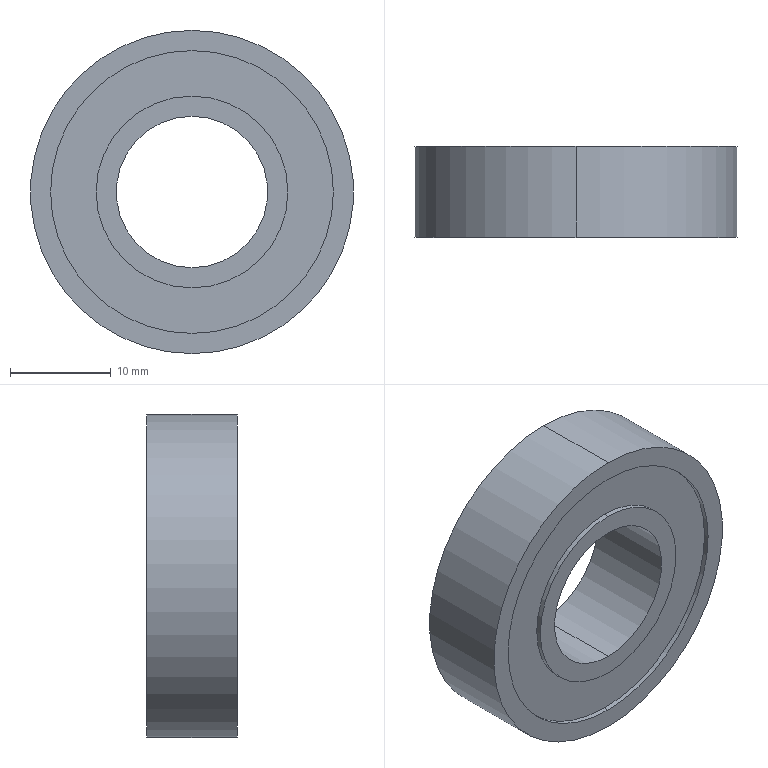Component | SolidWorks | 8TC-A15004-83-00-16_6002-2 | 1 solid | 18 faces | box 32 x 9 x 32 mm | volume 5316 mm3 | cylinder 12 | plane 6 | commonest cylinder face diameters 28 x4 19 x4 32 x2 15 x2
build123d program:
from build123d import *


with BuildPart() as part:
    # Sketch1 → Revolve1 (revolve)
    with BuildSketch(Plane(origin=(0, 0, 0), x_dir=(1, 0, 0), z_dir=(0, 1, 0)), mode=Mode.PRIVATE) as revolve1_sk:
        Polygon((-16, -4.5), (-16, 4.5), (-14, 4.5), (-14, 4), (-9.5, 4), (-9.5, 4.5), (-7.5, 4.5), (-7.5, -4.5), (-9.5, -4.5), (-9.5, -4), (-14, -4), (-14, -4.5), align=None)
    revolve(revolve1_sk.sketch.rotate(Axis((0, 0, 0), (0, 0, -1)), 180), axis=Axis((0, 0, 0), (0, 0, -1)))


solid = part.part

# Placed as in the assembly
solid = solid.moved(Location((40, 233, 60), (90, 0, 0)))
STEP:
#1=COLOUR_RGB('',0.7922,0.8196,0.9333);
#2=FILL_AREA_STYLE_COLOUR('',#1);
#3=FILL_AREA_STYLE('',(#2));
#4=SURFACE_STYLE_FILL_AREA(#3);
#5=SURFACE_SIDE_STYLE('',(#4));
#6=SURFACE_STYLE_USAGE(.BOTH.,#5);
#7=PRESENTATION_STYLE_ASSIGNMENT((#6));
#8=CARTESIAN_POINT('',(1.575,9.35,2.992));
#9=VERTEX_POINT('',#8);
#10=CARTESIAN_POINT('',(1.575,9.35,1.732));
#11=VERTEX_POINT('',#10);
#12=CARTESIAN_POINT('',(1.575,9.35,2.362));
#13=DIRECTION('',(-0.,-1.,0.));
#14=DIRECTION('',(0.,0.,1.));
#15=AXIS2_PLACEMENT_3D('',#12,#13,#14);
#16=CIRCLE('',#15,0.6299);
#17=EDGE_CURVE('',#9,#11,#16,.T.);
#18=ORIENTED_EDGE('',*,*,#17,.T.);
#19=CARTESIAN_POINT('',(1.575,8.996,1.732));
#20=VERTEX_POINT('',#19);
#21=CARTESIAN_POINT('',(1.575,9.173,1.732));
#22=DIRECTION('',(-0.,-1.,0.));
#23=VECTOR('',#22,39.37);
#24=LINE('',#21,#23);
#25=EDGE_CURVE('',#11,#20,#24,.T.);
#26=ORIENTED_EDGE('',*,*,#25,.T.);
#27=CARTESIAN_POINT('',(1.575,8.996,2.992));
#28=VERTEX_POINT('',#27);
#29=CARTESIAN_POINT('',(1.575,8.996,2.362));
#30=DIRECTION('',(-0.,-1.,0.));
#31=DIRECTION('',(0.,0.,1.));
#32=AXIS2_PLACEMENT_3D('',#29,#30,#31);
#33=CIRCLE('',#32,0.6299);
#34=EDGE_CURVE('',#28,#20,#33,.T.);
#35=ORIENTED_EDGE('',*,*,#34,.F.);
#36=CARTESIAN_POINT('',(1.575,9.173,2.992));
#37=DIRECTION('',(-0.,-1.,0.));
#38=VECTOR('',#37,39.37);
#39=LINE('',#36,#38);
#40=EDGE_CURVE('',#9,#28,#39,.T.);
#41=ORIENTED_EDGE('',*,*,#40,.F.);
#42=EDGE_LOOP('',(#18,#26,#35,#41));
#43=FACE_OUTER_BOUND('',#42,.T.);
#44=CARTESIAN_POINT('',(1.575,9.173,2.362));
#45=DIRECTION('',(-0.,-1.,0.));
#46=DIRECTION('',(0.,0.,1.));
#47=AXIS2_PLACEMENT_3D('',#44,#45,#46);
#48=CYLINDRICAL_SURFACE('',#47,0.6299);
#49=ADVANCED_FACE('',(#43),#48,.T.);
#50=CARTESIAN_POINT('',(1.575,9.016,1.811));
#51=VERTEX_POINT('',#50);
#52=CARTESIAN_POINT('',(1.575,9.016,2.913));
#53=VERTEX_POINT('',#52);
#54=CARTESIAN_POINT('',(1.575,9.016,2.362));
#55=DIRECTION('',(-0.,-1.,0.));
#56=DIRECTION('',(0.,0.,1.));
#57=AXIS2_PLACEMENT_3D('',#54,#55,#56);
#58=CIRCLE('',#57,0.5512);
#59=EDGE_CURVE('',#51,#53,#58,.T.);
#60=ORIENTED_EDGE('',*,*,#59,.F.);
#61=CARTESIAN_POINT('',(1.575,8.996,1.811));
#62=VERTEX_POINT('',#61);
#63=CARTESIAN_POINT('',(1.575,9.173,1.811));
#64=DIRECTION('',(-0.,-1.,0.));
#65=VECTOR('',#64,39.37);
#66=LINE('',#63,#65);
#67=EDGE_CURVE('',#51,#62,#66,.T.);
#68=ORIENTED_EDGE('',*,*,#67,.T.);
#69=CARTESIAN_POINT('',(1.575,8.996,2.913));
#70=VERTEX_POINT('',#69);
#71=CARTESIAN_POINT('',(1.575,8.996,2.362));
#72=DIRECTION('',(-0.,-1.,0.));
#73=DIRECTION('',(0.,0.,1.));
#74=AXIS2_PLACEMENT_3D('',#71,#72,#73);
#75=CIRCLE('',#74,0.5512);
#76=EDGE_CURVE('',#62,#70,#75,.T.);
#77=ORIENTED_EDGE('',*,*,#76,.T.);
#78=CARTESIAN_POINT('',(1.575,9.173,2.913));
#79=DIRECTION('',(-0.,-1.,0.));
#80=VECTOR('',#79,39.37);
#81=LINE('',#78,#80);
#82=EDGE_CURVE('',#53,#70,#81,.T.);
#83=ORIENTED_EDGE('',*,*,#82,.F.);
#84=EDGE_LOOP('',(#60,#68,#77,#83));
#85=FACE_OUTER_BOUND('',#84,.T.);
#86=CARTESIAN_POINT('',(1.575,9.173,2.362));
#87=DIRECTION('',(-0.,-1.,0.));
#88=DIRECTION('',(0.,0.,1.));
#89=AXIS2_PLACEMENT_3D('',#86,#87,#88);
#90=CYLINDRICAL_SURFACE('',#89,0.5512);
#91=ADVANCED_FACE('',(#85),#90,.F.);
#92=CARTESIAN_POINT('',(1.575,9.016,2.736));
#93=VERTEX_POINT('',#92);
#94=CARTESIAN_POINT('',(1.575,9.016,1.988));
#95=VERTEX_POINT('',#94);
#96=CARTESIAN_POINT('',(1.575,9.016,2.362));
#97=DIRECTION('',(-0.,-1.,0.));
#98=DIRECTION('',(0.,0.,1.));
#99=AXIS2_PLACEMENT_3D('',#96,#97,#98);
#100=CIRCLE('',#99,0.374);
#101=EDGE_CURVE('',#93,#95,#100,.T.);
#102=ORIENTED_EDGE('',*,*,#101,.T.);
#103=CARTESIAN_POINT('',(1.575,8.996,1.988));
#104=VERTEX_POINT('',#103);
#105=CARTESIAN_POINT('',(1.575,9.173,1.988));
#106=DIRECTION('',(-0.,-1.,0.));
#107=VECTOR('',#106,39.37);
#108=LINE('',#105,#107);
#109=EDGE_CURVE('',#95,#104,#108,.T.);
#110=ORIENTED_EDGE('',*,*,#109,.T.);
#111=CARTESIAN_POINT('',(1.575,8.996,2.736));
#112=VERTEX_POINT('',#111);
#113=CARTESIAN_POINT('',(1.575,8.996,2.362));
#114=DIRECTION('',(-0.,-1.,0.));
#115=DIRECTION('',(0.,0.,1.));
#116=AXIS2_PLACEMENT_3D('',#113,#114,#115);
#117=CIRCLE('',#116,0.374);
#118=EDGE_CURVE('',#112,#104,#117,.T.);
#119=ORIENTED_EDGE('',*,*,#118,.F.);
#120=CARTESIAN_POINT('',(1.575,9.173,2.736));
#121=DIRECTION('',(-0.,-1.,0.));
#122=VECTOR('',#121,39.37);
#123=LINE('',#120,#122);
#124=EDGE_CURVE('',#93,#112,#123,.T.);
#125=ORIENTED_EDGE('',*,*,#124,.F.);
#126=EDGE_LOOP('',(#102,#110,#119,#125));
#127=FACE_OUTER_BOUND('',#126,.T.);
#128=CARTESIAN_POINT('',(1.575,9.173,2.362));
#129=DIRECTION('',(-0.,-1.,0.));
#130=DIRECTION('',(0.,0.,1.));
#131=AXIS2_PLACEMENT_3D('',#128,#129,#130);
#132=CYLINDRICAL_SURFACE('',#131,0.374);
#133=ADVANCED_FACE('',(#127),#132,.T.);
#134=CARTESIAN_POINT('',(1.575,9.35,2.067));
#135=VERTEX_POINT('',#134);
#136=CARTESIAN_POINT('',(1.575,9.35,2.657));
#137=VERTEX_POINT('',#136);
#138=CARTESIAN_POINT('',(1.575,9.35,2.362));
#139=DIRECTION('',(-0.,-1.,0.));
#140=DIRECTION('',(0.,0.,1.));
#141=AXIS2_PLACEMENT_3D('',#138,#139,#140);
#142=CIRCLE('',#141,0.2953);
#143=EDGE_CURVE('',#135,#137,#142,.T.);
#144=ORIENTED_EDGE('',*,*,#143,.F.);
#145=CARTESIAN_POINT('',(1.575,8.996,2.067));
#146=VERTEX_POINT('',#145);
#147=CARTESIAN_POINT('',(1.575,9.173,2.067));
#148=DIRECTION('',(-0.,-1.,0.));
#149=VECTOR('',#148,39.37);
#150=LINE('',#147,#149);
#151=EDGE_CURVE('',#135,#146,#150,.T.);
#152=ORIENTED_EDGE('',*,*,#151,.T.);
#153=CARTESIAN_POINT('',(1.575,8.996,2.657));
#154=VERTEX_POINT('',#153);
#155=CARTESIAN_POINT('',(1.575,8.996,2.362));
#156=DIRECTION('',(-0.,-1.,0.));
#157=DIRECTION('',(0.,0.,1.));
#158=AXIS2_PLACEMENT_3D('',#155,#156,#157);
#159=CIRCLE('',#158,0.2953);
#160=EDGE_CURVE('',#146,#154,#159,.T.);
#161=ORIENTED_EDGE('',*,*,#160,.T.);
#162=CARTESIAN_POINT('',(1.575,9.173,2.657));
#163=DIRECTION('',(-0.,-1.,0.));
#164=VECTOR('',#163,39.37);
#165=LINE('',#162,#164);
#166=EDGE_CURVE('',#137,#154,#165,.T.);
#167=ORIENTED_EDGE('',*,*,#166,.F.);
#168=EDGE_LOOP('',(#144,#152,#161,#167));
#169=FACE_OUTER_BOUND('',#168,.T.);
#170=CARTESIAN_POINT('',(1.575,9.173,2.362));
#171=DIRECTION('',(-0.,-1.,0.));
#172=DIRECTION('',(0.,0.,1.));
#173=AXIS2_PLACEMENT_3D('',#170,#171,#172);
#174=CYLINDRICAL_SURFACE('',#173,0.2953);
#175=ADVANCED_FACE('',(#169),#174,.F.);
#176=CARTESIAN_POINT('',(1.575,9.35,2.736));
#177=VERTEX_POINT('',#176);
#178=CARTESIAN_POINT('',(1.575,9.35,1.988));
#179=VERTEX_POINT('',#178);
#180=CARTESIAN_POINT('',(1.575,9.35,2.362));
#181=DIRECTION('',(-0.,-1.,0.));
#182=DIRECTION('',(0.,0.,1.));
#183=AXIS2_PLACEMENT_3D('',#180,#181,#182);
#184=CIRCLE('',#183,0.374);
#185=EDGE_CURVE('',#177,#179,#184,.T.);
#186=ORIENTED_EDGE('',*,*,#185,.T.);
#187=CARTESIAN_POINT('',(1.575,9.331,1.988));
#188=VERTEX_POINT('',#187);
#189=CARTESIAN_POINT('',(1.575,9.173,1.988));
#190=DIRECTION('',(-0.,-1.,0.));
#191=VECTOR('',#190,39.37);
#192=LINE('',#189,#191);
#193=EDGE_CURVE('',#179,#188,#192,.T.);
#194=ORIENTED_EDGE('',*,*,#193,.T.);
#195=CARTESIAN_POINT('',(1.575,9.331,2.736));
#196=VERTEX_POINT('',#195);
#197=CARTESIAN_POINT('',(1.575,9.331,2.362));
#198=DIRECTION('',(-0.,-1.,0.));
#199=DIRECTION('',(0.,0.,1.));
#200=AXIS2_PLACEMENT_3D('',#197,#198,#199);
#201=CIRCLE('',#200,0.374);
#202=EDGE_CURVE('',#196,#188,#201,.T.);
#203=ORIENTED_EDGE('',*,*,#202,.F.);
#204=CARTESIAN_POINT('',(1.575,9.173,2.736));
#205=DIRECTION('',(-0.,-1.,0.));
#206=VECTOR('',#205,39.37);
#207=LINE('',#204,#206);
#208=EDGE_CURVE('',#177,#196,#207,.T.);
#209=ORIENTED_EDGE('',*,*,#208,.F.);
#210=EDGE_LOOP('',(#186,#194,#203,#209));
#211=FACE_OUTER_BOUND('',#210,.T.);
#212=CARTESIAN_POINT('',(1.575,9.173,2.362));
#213=DIRECTION('',(-0.,-1.,0.));
#214=DIRECTION('',(0.,0.,1.));
#215=AXIS2_PLACEMENT_3D('',#212,#213,#214);
#216=CYLINDRICAL_SURFACE('',#215,0.374);
#217=ADVANCED_FACE('',(#211),#216,.T.);
#218=CARTESIAN_POINT('',(1.575,9.35,1.811));
#219=VERTEX_POINT('',#218);
#220=CARTESIAN_POINT('',(1.575,9.35,2.913));
#221=VERTEX_POINT('',#220);
#222=CARTESIAN_POINT('',(1.575,9.35,2.362));
#223=DIRECTION('',(-0.,-1.,0.));
#224=DIRECTION('',(0.,0.,1.));
#225=AXIS2_PLACEMENT_3D('',#222,#223,#224);
#226=CIRCLE('',#225,0.5512);
#227=EDGE_CURVE('',#219,#221,#226,.T.);
#228=ORIENTED_EDGE('',*,*,#227,.F.);
#229=CARTESIAN_POINT('',(1.575,9.331,1.811));
#230=VERTEX_POINT('',#229);
#231=CARTESIAN_POINT('',(1.575,9.173,1.811));
#232=DIRECTION('',(-0.,-1.,0.));
#233=VECTOR('',#232,39.37);
#234=LINE('',#231,#233);
#235=EDGE_CURVE('',#219,#230,#234,.T.);
#236=ORIENTED_EDGE('',*,*,#235,.T.);
#237=CARTESIAN_POINT('',(1.575,9.331,2.913));
#238=VERTEX_POINT('',#237);
#239=CARTESIAN_POINT('',(1.575,9.331,2.362));
#240=DIRECTION('',(-0.,-1.,0.));
#241=DIRECTION('',(0.,0.,1.));
#242=AXIS2_PLACEMENT_3D('',#239,#240,#241);
#243=CIRCLE('',#242,0.5512);
#244=EDGE_CURVE('',#230,#238,#243,.T.);
#245=ORIENTED_EDGE('',*,*,#244,.T.);
#246=CARTESIAN_POINT('',(1.575,9.173,2.913));
#247=DIRECTION('',(-0.,-1.,0.));
#248=VECTOR('',#247,39.37);
#249=LINE('',#246,#248);
#250=EDGE_CURVE('',#221,#238,#249,.T.);
#251=ORIENTED_EDGE('',*,*,#250,.F.);
#252=EDGE_LOOP('',(#228,#236,#245,#251));
#253=FACE_OUTER_BOUND('',#252,.T.);
#254=CARTESIAN_POINT('',(1.575,9.173,2.362));
#255=DIRECTION('',(-0.,-1.,0.));
#256=DIRECTION('',(0.,0.,1.));
#257=AXIS2_PLACEMENT_3D('',#254,#255,#256);
#258=CYLINDRICAL_SURFACE('',#257,0.5512);
#259=ADVANCED_FACE('',(#253),#258,.F.);
#260=ORIENTED_EDGE('',*,*,#17,.F.);
#261=CARTESIAN_POINT('',(1.575,9.35,2.362));
#262=DIRECTION('',(-0.,-1.,0.));
#263=DIRECTION('',(0.,0.,1.));
#264=AXIS2_PLACEMENT_3D('',#261,#262,#263);
#265=CIRCLE('',#264,0.6299);
#266=EDGE_CURVE('',#11,#9,#265,.T.);
#267=ORIENTED_EDGE('',*,*,#266,.F.);
#268=EDGE_LOOP('',(#260,#267));
#269=FACE_OUTER_BOUND('',#268,.T.);
#270=CARTESIAN_POINT('',(1.575,9.35,2.362));
#271=DIRECTION('',(-0.,-1.,0.));
#272=DIRECTION('',(0.,0.,1.));
#273=AXIS2_PLACEMENT_3D('',#270,#271,#272);
#274=CIRCLE('',#273,0.5512);
#275=EDGE_CURVE('',#221,#219,#274,.T.);
#276=ORIENTED_EDGE('',*,*,#275,.T.);
#277=ORIENTED_EDGE('',*,*,#227,.T.);
#278=EDGE_LOOP('',(#276,#277));
#279=FACE_BOUND('',#278,.T.);
#280=CARTESIAN_POINT('',(1.575,9.35,1.732));
#281=DIRECTION('',(-0.,-1.,0.));
#282=DIRECTION('',(0.,0.,1.));
#283=AXIS2_PLACEMENT_3D('',#280,#281,#282);
#284=PLANE('',#283);
#285=ADVANCED_FACE('',(#269,#279),#284,.F.);
#286=ORIENTED_EDGE('',*,*,#235,.F.);
#287=ORIENTED_EDGE('',*,*,#275,.F.);
#288=ORIENTED_EDGE('',*,*,#250,.T.);
#289=CARTESIAN_POINT('',(1.575,9.331,2.362));
#290=DIRECTION('',(-0.,-1.,0.));
#291=DIRECTION('',(0.,0.,1.));
#292=AXIS2_PLACEMENT_3D('',#289,#290,#291);
#293=CIRCLE('',#292,0.5512);
#294=EDGE_CURVE('',#238,#230,#293,.T.);
#295=ORIENTED_EDGE('',*,*,#294,.T.);
#296=EDGE_LOOP('',(#286,#287,#288,#295));
#297=FACE_OUTER_BOUND('',#296,.T.);
#298=CARTESIAN_POINT('',(1.575,9.173,2.362));
#299=DIRECTION('',(-0.,-1.,0.));
#300=DIRECTION('',(0.,0.,1.));
#301=AXIS2_PLACEMENT_3D('',#298,#299,#300);
#302=CYLINDRICAL_SURFACE('',#301,0.5512);
#303=ADVANCED_FACE('',(#297),#302,.F.);
#304=ORIENTED_EDGE('',*,*,#294,.F.);
#305=ORIENTED_EDGE('',*,*,#244,.F.);
#306=EDGE_LOOP('',(#304,#305));
#307=FACE_OUTER_BOUND('',#306,.T.);
#308=ORIENTED_EDGE('',*,*,#202,.T.);
#309=CARTESIAN_POINT('',(1.575,9.331,2.362));
#310=DIRECTION('',(-0.,-1.,0.));
#311=DIRECTION('',(0.,0.,1.));
#312=AXIS2_PLACEMENT_3D('',#309,#310,#311);
#313=CIRCLE('',#312,0.374);
#314=EDGE_CURVE('',#188,#196,#313,.T.);
#315=ORIENTED_EDGE('',*,*,#314,.T.);
#316=EDGE_LOOP('',(#308,#315));
#317=FACE_BOUND('',#316,.T.);
#318=CARTESIAN_POINT('',(1.575,9.331,1.811));
#319=DIRECTION('',(-0.,-1.,0.));
#320=DIRECTION('',(0.,0.,1.));
#321=AXIS2_PLACEMENT_3D('',#318,#319,#320);
#322=PLANE('',#321);
#323=ADVANCED_FACE('',(#307,#317),#322,.F.);
#324=ORIENTED_EDGE('',*,*,#193,.F.);
#325=CARTESIAN_POINT('',(1.575,9.35,2.362));
#326=DIRECTION('',(-0.,-1.,0.));
#327=DIRECTION('',(0.,0.,1.));
#328=AXIS2_PLACEMENT_3D('',#325,#326,#327);
#329=CIRCLE('',#328,0.374);
#330=EDGE_CURVE('',#179,#177,#329,.T.);
#331=ORIENTED_EDGE('',*,*,#330,.T.);
#332=ORIENTED_EDGE('',*,*,#208,.T.);
#333=ORIENTED_EDGE('',*,*,#314,.F.);
#334=EDGE_LOOP('',(#324,#331,#332,#333));
#335=FACE_OUTER_BOUND('',#334,.T.);
#336=CARTESIAN_POINT('',(1.575,9.173,2.362));
#337=DIRECTION('',(-0.,-1.,0.));
#338=DIRECTION('',(0.,0.,1.));
#339=AXIS2_PLACEMENT_3D('',#336,#337,#338);
#340=CYLINDRICAL_SURFACE('',#339,0.374);
#341=ADVANCED_FACE('',(#335),#340,.T.);
#342=ORIENTED_EDGE('',*,*,#185,.F.);
#343=ORIENTED_EDGE('',*,*,#330,.F.);
#344=EDGE_LOOP('',(#342,#343));
#345=FACE_OUTER_BOUND('',#344,.T.);
#346=CARTESIAN_POINT('',(1.575,9.35,2.362));
#347=DIRECTION('',(-0.,-1.,0.));
#348=DIRECTION('',(0.,0.,1.));
#349=AXIS2_PLACEMENT_3D('',#346,#347,#348);
#350=CIRCLE('',#349,0.2953);
#351=EDGE_CURVE('',#137,#135,#350,.T.);
#352=ORIENTED_EDGE('',*,*,#351,.T.);
#353=ORIENTED_EDGE('',*,*,#143,.T.);
#354=EDGE_LOOP('',(#352,#353));
#355=FACE_BOUND('',#354,.T.);
#356=CARTESIAN_POINT('',(1.575,9.35,1.988));
#357=DIRECTION('',(-0.,-1.,0.));
#358=DIRECTION('',(0.,0.,1.));
#359=AXIS2_PLACEMENT_3D('',#356,#357,#358);
#360=PLANE('',#359);
#361=ADVANCED_FACE('',(#345,#355),#360,.F.);
#362=ORIENTED_EDGE('',*,*,#151,.F.);
#363=ORIENTED_EDGE('',*,*,#351,.F.);
#364=ORIENTED_EDGE('',*,*,#166,.T.);
#365=CARTESIAN_POINT('',(1.575,8.996,2.362));
#366=DIRECTION('',(-0.,-1.,0.));
#367=DIRECTION('',(0.,0.,1.));
#368=AXIS2_PLACEMENT_3D('',#365,#366,#367);
#369=CIRCLE('',#368,0.2953);
#370=EDGE_CURVE('',#154,#146,#369,.T.);
#371=ORIENTED_EDGE('',*,*,#370,.T.);
#372=EDGE_LOOP('',(#362,#363,#364,#371));
#373=FACE_OUTER_BOUND('',#372,.T.);
#374=CARTESIAN_POINT('',(1.575,9.173,2.362));
#375=DIRECTION('',(-0.,-1.,0.));
#376=DIRECTION('',(0.,0.,1.));
#377=AXIS2_PLACEMENT_3D('',#374,#375,#376);
#378=CYLINDRICAL_SURFACE('',#377,0.2953);
#379=ADVANCED_FACE('',(#373),#378,.F.);
#380=ORIENTED_EDGE('',*,*,#370,.F.);
#381=ORIENTED_EDGE('',*,*,#160,.F.);
#382=EDGE_LOOP('',(#380,#381));
#383=FACE_BOUND('',#382,.T.);
#384=ORIENTED_EDGE('',*,*,#118,.T.);
#385=CARTESIAN_POINT('',(1.575,8.996,2.362));
#386=DIRECTION('',(-0.,-1.,0.));
#387=DIRECTION('',(0.,0.,1.));
#388=AXIS2_PLACEMENT_3D('',#385,#386,#387);
#389=CIRCLE('',#388,0.374);
#390=EDGE_CURVE('',#104,#112,#389,.T.);
#391=ORIENTED_EDGE('',*,*,#390,.T.);
#392=EDGE_LOOP('',(#384,#391));
#393=FACE_OUTER_BOUND('',#392,.T.);
#394=CARTESIAN_POINT('',(1.575,8.996,1.988));
#395=DIRECTION('',(0.,1.,0.));
#396=DIRECTION('',(0.,0.,-1.));
#397=AXIS2_PLACEMENT_3D('',#394,#395,#396);
#398=PLANE('',#397);
#399=ADVANCED_FACE('',(#383,#393),#398,.F.);
#400=ORIENTED_EDGE('',*,*,#109,.F.);
#401=CARTESIAN_POINT('',(1.575,9.016,2.362));
#402=DIRECTION('',(-0.,-1.,0.));
#403=DIRECTION('',(0.,0.,1.));
#404=AXIS2_PLACEMENT_3D('',#401,#402,#403);
#405=CIRCLE('',#404,0.374);
#406=EDGE_CURVE('',#95,#93,#405,.T.);
#407=ORIENTED_EDGE('',*,*,#406,.T.);
#408=ORIENTED_EDGE('',*,*,#124,.T.);
#409=ORIENTED_EDGE('',*,*,#390,.F.);
#410=EDGE_LOOP('',(#400,#407,#408,#409));
#411=FACE_OUTER_BOUND('',#410,.T.);
#412=CARTESIAN_POINT('',(1.575,9.173,2.362));
#413=DIRECTION('',(-0.,-1.,0.));
#414=DIRECTION('',(0.,0.,1.));
#415=AXIS2_PLACEMENT_3D('',#412,#413,#414);
#416=CYLINDRICAL_SURFACE('',#415,0.374);
#417=ADVANCED_FACE('',(#411),#416,.T.);
#418=ORIENTED_EDGE('',*,*,#101,.F.);
#419=ORIENTED_EDGE('',*,*,#406,.F.);
#420=EDGE_LOOP('',(#418,#419));
#421=FACE_BOUND('',#420,.T.);
#422=CARTESIAN_POINT('',(1.575,9.016,2.362));
#423=DIRECTION('',(-0.,-1.,0.));
#424=DIRECTION('',(0.,0.,1.));
#425=AXIS2_PLACEMENT_3D('',#422,#423,#424);
#426=CIRCLE('',#425,0.5512);
#427=EDGE_CURVE('',#53,#51,#426,.T.);
#428=ORIENTED_EDGE('',*,*,#427,.T.);
#429=ORIENTED_EDGE('',*,*,#59,.T.);
#430=EDGE_LOOP('',(#428,#429));
#431=FACE_OUTER_BOUND('',#430,.T.);
#432=CARTESIAN_POINT('',(1.575,9.016,1.811));
#433=DIRECTION('',(0.,1.,0.));
#434=DIRECTION('',(0.,0.,-1.));
#435=AXIS2_PLACEMENT_3D('',#432,#433,#434);
#436=PLANE('',#435);
#437=ADVANCED_FACE('',(#421,#431),#436,.F.);
#438=ORIENTED_EDGE('',*,*,#67,.F.);
#439=ORIENTED_EDGE('',*,*,#427,.F.);
#440=ORIENTED_EDGE('',*,*,#82,.T.);
#441=CARTESIAN_POINT('',(1.575,8.996,2.362));
#442=DIRECTION('',(-0.,-1.,0.));
#443=DIRECTION('',(0.,0.,1.));
#444=AXIS2_PLACEMENT_3D('',#441,#442,#443);
#445=CIRCLE('',#444,0.5512);
#446=EDGE_CURVE('',#70,#62,#445,.T.);
#447=ORIENTED_EDGE('',*,*,#446,.T.);
#448=EDGE_LOOP('',(#438,#439,#440,#447));
#449=FACE_OUTER_BOUND('',#448,.T.);
#450=CARTESIAN_POINT('',(1.575,9.173,2.362));
#451=DIRECTION('',(-0.,-1.,0.));
#452=DIRECTION('',(0.,0.,1.));
#453=AXIS2_PLACEMENT_3D('',#450,#451,#452);
#454=CYLINDRICAL_SURFACE('',#453,0.5512);
#455=ADVANCED_FACE('',(#449),#454,.F.);
#456=ORIENTED_EDGE('',*,*,#446,.F.);
#457=ORIENTED_EDGE('',*,*,#76,.F.);
#458=EDGE_LOOP('',(#456,#457));
#459=FACE_BOUND('',#458,.T.);
#460=ORIENTED_EDGE('',*,*,#34,.T.);
#461=CARTESIAN_POINT('',(1.575,8.996,2.362));
#462=DIRECTION('',(-0.,-1.,0.));
#463=DIRECTION('',(0.,0.,1.));
#464=AXIS2_PLACEMENT_3D('',#461,#462,#463);
#465=CIRCLE('',#464,0.6299);
#466=EDGE_CURVE('',#20,#28,#465,.T.);
#467=ORIENTED_EDGE('',*,*,#466,.T.);
#468=EDGE_LOOP('',(#460,#467));
#469=FACE_OUTER_BOUND('',#468,.T.);
#470=CARTESIAN_POINT('',(1.575,8.996,1.732));
#471=DIRECTION('',(0.,1.,0.));
#472=DIRECTION('',(0.,0.,-1.));
#473=AXIS2_PLACEMENT_3D('',#470,#471,#472);
#474=PLANE('',#473);
#475=ADVANCED_FACE('',(#459,#469),#474,.F.);
#476=ORIENTED_EDGE('',*,*,#25,.F.);
#477=ORIENTED_EDGE('',*,*,#266,.T.);
#478=ORIENTED_EDGE('',*,*,#40,.T.);
#479=ORIENTED_EDGE('',*,*,#466,.F.);
#480=EDGE_LOOP('',(#476,#477,#478,#479));
#481=FACE_OUTER_BOUND('',#480,.T.);
#482=CARTESIAN_POINT('',(1.575,9.173,2.362));
#483=DIRECTION('',(-0.,-1.,0.));
#484=DIRECTION('',(0.,0.,1.));
#485=AXIS2_PLACEMENT_3D('',#482,#483,#484);
#486=CYLINDRICAL_SURFACE('',#485,0.6299);
#487=ADVANCED_FACE('',(#481),#486,.T.);
#488=CLOSED_SHELL('',(#49,#91,#133,#175,#217,#259,#285,#303,#323,#341,#361,#379,#399,#417,#437,#455,#475,#487));
#489=MANIFOLD_SOLID_BREP('',#488);
#490=STYLED_ITEM('',(#7),#489);
#491=PRESENTATION_LAYER_ASSIGNMENT('','',(#490));
#492=CARTESIAN_POINT('',(0.,0.,0.));
#493=DIRECTION('',(0.,0.,1.));
#494=DIRECTION('',(1.,0.,0.));
#495=AXIS2_PLACEMENT_3D('',#492,#493,#494);
#496=(LENGTH_UNIT()NAMED_UNIT(*)SI_UNIT($,.METRE.));
#497=LENGTH_MEASURE_WITH_UNIT(LENGTH_MEASURE(0.0254),#496);
#498=DIMENSIONAL_EXPONENTS(1.,0.,0.,0.,0.,0.,0.);
#499=(CONVERSION_BASED_UNIT('',#497)LENGTH_UNIT()NAMED_UNIT(#498));
#500=UNCERTAINTY_MEASURE_WITH_UNIT(LENGTH_MEASURE(0.00001),#499,'','');
#501=(NAMED_UNIT(*)PLANE_ANGLE_UNIT()SI_UNIT($,.RADIAN.));
#502=(NAMED_UNIT(*)SI_UNIT($,.STERADIAN.)SOLID_ANGLE_UNIT());
#503=(GEOMETRIC_REPRESENTATION_CONTEXT(3)GLOBAL_UNCERTAINTY_ASSIGNED_CONTEXT((#500))GLOBAL_UNIT_ASSIGNED_CONTEXT((#499,#501,#502))REPRESENTATION_CONTEXT('',''));
#504=ADVANCED_BREP_SHAPE_REPRESENTATION('',(#489,#495),#503);
#505=(LENGTH_UNIT()NAMED_UNIT(*)SI_UNIT($,.METRE.));
#506=LENGTH_MEASURE_WITH_UNIT(LENGTH_MEASURE(0.0254),#505);
#507=DIMENSIONAL_EXPONENTS(1.,0.,0.,0.,0.,0.,0.);
#508=(CONVERSION_BASED_UNIT('',#506)LENGTH_UNIT()NAMED_UNIT(#507));
#509=UNCERTAINTY_MEASURE_WITH_UNIT(LENGTH_MEASURE(0.00001),#508,'','');
#510=(NAMED_UNIT(*)PLANE_ANGLE_UNIT()SI_UNIT($,.RADIAN.));
#511=(NAMED_UNIT(*)SI_UNIT($,.STERADIAN.)SOLID_ANGLE_UNIT());
#512=(GEOMETRIC_REPRESENTATION_CONTEXT(3)GLOBAL_UNCERTAINTY_ASSIGNED_CONTEXT((#509))GLOBAL_UNIT_ASSIGNED_CONTEXT((#508,#510,#511))REPRESENTATION_CONTEXT('',''));
#513=MECHANICAL_DESIGN_GEOMETRIC_PRESENTATION_REPRESENTATION('',(#490),#512);